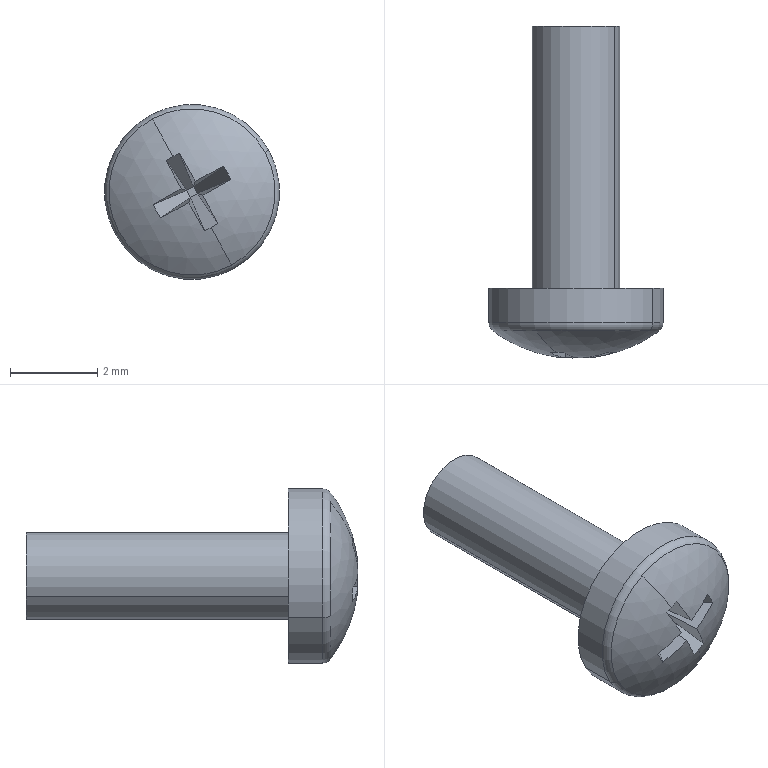Component | SolidWorks | pan cross head_am_pkg-24 | 1 solid | 23 faces | box 4 x 7.59 x 4 mm | volume 34 mm3 | plane 15 | cylinder 4 | torus 2 | sphere 2 | commonest cylinder face diameters 4 x2 2 x2
STEP:
#1=COLOUR_RGB('',0.7922,0.8196,0.9333);
#2=FILL_AREA_STYLE_COLOUR('',#1);
#3=FILL_AREA_STYLE('',(#2));
#4=SURFACE_STYLE_FILL_AREA(#3);
#5=SURFACE_SIDE_STYLE('',(#4));
#6=SURFACE_STYLE_USAGE(.BOTH.,#5);
#7=PRESENTATION_STYLE_ASSIGNMENT((#6));
#8=CARTESIAN_POINT('',(-3.41,0.1268,3.067));
#9=VERTEX_POINT('',#8);
#10=CARTESIAN_POINT('',(-3.271,0.1268,3.142));
#11=VERTEX_POINT('',#10);
#12=CARTESIAN_POINT('',(-3.341,0.1268,3.104));
#13=DIRECTION('',(0.,-1.,0.));
#14=DIRECTION('',(-0.8793,0.,-0.4763));
#15=AXIS2_PLACEMENT_3D('',#12,#13,#14);
#16=CIRCLE('',#15,0.07874);
#17=EDGE_CURVE('',#9,#11,#16,.T.);
#18=ORIENTED_EDGE('',*,*,#17,.T.);
#19=CARTESIAN_POINT('',(-3.275,0.1192,3.14));
#20=VERTEX_POINT('',#19);
#21=CARTESIAN_POINT('',(-3.28,0.1268,3.137));
#22=DIRECTION('',(0.4763,0.,-0.8793));
#23=DIRECTION('',(-0.8793,0.,-0.4763));
#24=AXIS2_PLACEMENT_3D('',#21,#22,#23);
#25=CIRCLE('',#24,0.009449);
#26=EDGE_CURVE('',#11,#20,#25,.T.);
#27=ORIENTED_EDGE('',*,*,#26,.T.);
#28=CARTESIAN_POINT('',(-3.305,0.1192,3.039));
#29=VERTEX_POINT('',#28);
#30=CARTESIAN_POINT('',(-3.341,0.1192,3.104));
#31=DIRECTION('',(0.,-1.,0.));
#32=DIRECTION('',(-0.8793,0.,-0.4763));
#33=AXIS2_PLACEMENT_3D('',#30,#31,#32);
#34=CIRCLE('',#33,0.07491);
#35=EDGE_CURVE('',#29,#20,#34,.T.);
#36=ORIENTED_EDGE('',*,*,#35,.F.);
#37=CARTESIAN_POINT('',(-3.407,0.1192,3.069));
#38=VERTEX_POINT('',#37);
#39=CARTESIAN_POINT('',(-3.341,0.1192,3.104));
#40=DIRECTION('',(0.,-1.,0.));
#41=DIRECTION('',(-0.8793,0.,-0.4763));
#42=AXIS2_PLACEMENT_3D('',#39,#40,#41);
#43=CIRCLE('',#42,0.07491);
#44=EDGE_CURVE('',#38,#29,#43,.T.);
#45=ORIENTED_EDGE('',*,*,#44,.F.);
#46=CARTESIAN_POINT('',(-3.402,0.1268,3.071));
#47=DIRECTION('',(-0.4763,0.,0.8793));
#48=DIRECTION('',(0.8793,0.,0.4763));
#49=AXIS2_PLACEMENT_3D('',#46,#47,#48);
#50=CIRCLE('',#49,0.009449);
#51=EDGE_CURVE('',#9,#38,#50,.T.);
#52=ORIENTED_EDGE('',*,*,#51,.F.);
#53=EDGE_LOOP('',(#18,#27,#36,#45,#52));
#54=FACE_OUTER_BOUND('',#53,.T.);
#55=CARTESIAN_POINT('',(-3.341,0.1268,3.104));
#56=DIRECTION('',(0.,-1.,0.));
#57=DIRECTION('',(-0.8793,0.,-0.4763));
#58=AXIS2_PLACEMENT_3D('',#55,#56,#57);
#59=TOROIDAL_SURFACE('',#58,0.06929,0.009449);
#60=ADVANCED_FACE('',(#54),#59,.T.);
#61=CARTESIAN_POINT('',(-3.41,0.1575,3.067));
#62=VERTEX_POINT('',#61);
#63=CARTESIAN_POINT('',(-3.271,0.1575,3.142));
#64=VERTEX_POINT('',#63);
#65=CARTESIAN_POINT('',(-3.341,0.1575,3.104));
#66=DIRECTION('',(0.,-1.,0.));
#67=DIRECTION('',(-0.8793,0.,-0.4763));
#68=AXIS2_PLACEMENT_3D('',#65,#66,#67);
#69=CIRCLE('',#68,0.07874);
#70=EDGE_CURVE('',#62,#64,#69,.T.);
#71=ORIENTED_EDGE('',*,*,#70,.T.);
#72=CARTESIAN_POINT('',(-3.271,-0.9055,3.142));
#73=DIRECTION('',(0.,-1.,0.));
#74=VECTOR('',#73,39.37);
#75=LINE('',#72,#74);
#76=EDGE_CURVE('',#64,#11,#75,.T.);
#77=ORIENTED_EDGE('',*,*,#76,.T.);
#78=ORIENTED_EDGE('',*,*,#17,.F.);
#79=CARTESIAN_POINT('',(-3.41,-0.9055,3.067));
#80=DIRECTION('',(0.,-1.,0.));
#81=VECTOR('',#80,39.37);
#82=LINE('',#79,#81);
#83=EDGE_CURVE('',#62,#9,#82,.T.);
#84=ORIENTED_EDGE('',*,*,#83,.F.);
#85=EDGE_LOOP('',(#71,#77,#78,#84));
#86=FACE_OUTER_BOUND('',#85,.T.);
#87=CARTESIAN_POINT('',(-3.341,-0.9055,3.104));
#88=DIRECTION('',(0.,-1.,0.));
#89=DIRECTION('',(-0.8793,0.,-0.4763));
#90=AXIS2_PLACEMENT_3D('',#87,#88,#89);
#91=CYLINDRICAL_SURFACE('',#90,0.07874);
#92=ADVANCED_FACE('',(#86),#91,.T.);
#93=CARTESIAN_POINT('',(-3.375,0.3937,3.086));
#94=VERTEX_POINT('',#93);
#95=CARTESIAN_POINT('',(-3.306,0.3937,3.123));
#96=VERTEX_POINT('',#95);
#97=CARTESIAN_POINT('',(-3.341,0.3937,3.104));
#98=DIRECTION('',(0.,-1.,0.));
#99=DIRECTION('',(-0.8793,0.,-0.4763));
#100=AXIS2_PLACEMENT_3D('',#97,#98,#99);
#101=CIRCLE('',#100,0.03937);
#102=EDGE_CURVE('',#94,#96,#101,.T.);
#103=ORIENTED_EDGE('',*,*,#102,.T.);
#104=CARTESIAN_POINT('',(-3.306,0.1575,3.123));
#105=VERTEX_POINT('',#104);
#106=CARTESIAN_POINT('',(-3.306,-0.9055,3.123));
#107=DIRECTION('',(0.,-1.,0.));
#108=VECTOR('',#107,39.37);
#109=LINE('',#106,#108);
#110=EDGE_CURVE('',#96,#105,#109,.T.);
#111=ORIENTED_EDGE('',*,*,#110,.T.);
#112=CARTESIAN_POINT('',(-3.375,0.1575,3.086));
#113=VERTEX_POINT('',#112);
#114=CARTESIAN_POINT('',(-3.341,0.1575,3.104));
#115=DIRECTION('',(0.,-1.,0.));
#116=DIRECTION('',(-0.8793,0.,-0.4763));
#117=AXIS2_PLACEMENT_3D('',#114,#115,#116);
#118=CIRCLE('',#117,0.03937);
#119=EDGE_CURVE('',#113,#105,#118,.T.);
#120=ORIENTED_EDGE('',*,*,#119,.F.);
#121=CARTESIAN_POINT('',(-3.375,-0.9055,3.086));
#122=DIRECTION('',(0.,-1.,0.));
#123=VECTOR('',#122,39.37);
#124=LINE('',#121,#123);
#125=EDGE_CURVE('',#94,#113,#124,.T.);
#126=ORIENTED_EDGE('',*,*,#125,.F.);
#127=EDGE_LOOP('',(#103,#111,#120,#126));
#128=FACE_OUTER_BOUND('',#127,.T.);
#129=CARTESIAN_POINT('',(-3.341,-0.9055,3.104));
#130=DIRECTION('',(0.,-1.,0.));
#131=DIRECTION('',(-0.8793,0.,-0.4763));
#132=AXIS2_PLACEMENT_3D('',#129,#130,#131);
#133=CYLINDRICAL_SURFACE('',#132,0.03937);
#134=ADVANCED_FACE('',(#128),#133,.T.);
#135=ORIENTED_EDGE('',*,*,#35,.T.);
#136=CARTESIAN_POINT('',(-3.376,0.1192,3.17));
#137=VERTEX_POINT('',#136);
#138=CARTESIAN_POINT('',(-3.341,0.1192,3.104));
#139=DIRECTION('',(0.,-1.,0.));
#140=DIRECTION('',(-0.8793,0.,-0.4763));
#141=AXIS2_PLACEMENT_3D('',#138,#139,#140);
#142=CIRCLE('',#141,0.07491);
#143=EDGE_CURVE('',#20,#137,#142,.T.);
#144=ORIENTED_EDGE('',*,*,#143,.T.);
#145=CARTESIAN_POINT('',(-3.358,0.09982,3.136));
#146=VERTEX_POINT('',#145);
#147=CARTESIAN_POINT('',(-3.341,0.2205,3.104));
#148=DIRECTION('',(0.8793,0.,0.4763));
#149=DIRECTION('',(0.4763,0.,-0.8793));
#150=AXIS2_PLACEMENT_3D('',#147,#148,#149);
#151=CIRCLE('',#150,0.126);
#152=EDGE_CURVE('',#137,#146,#151,.T.);
#153=ORIENTED_EDGE('',*,*,#152,.T.);
#154=CARTESIAN_POINT('',(-3.352,0.09998,3.14));
#155=VERTEX_POINT('',#154);
#156=CARTESIAN_POINT('',(-3.325,0.197,3.075));
#157=DIRECTION('',(-0.3878,0.5805,0.716));
#158=DIRECTION('',(0.2765,0.8143,-0.5104));
#159=AXIS2_PLACEMENT_3D('',#156,#157,#158);
#160=CIRCLE('',#159,0.1193);
#161=EDGE_CURVE('',#146,#155,#160,.T.);
#162=ORIENTED_EDGE('',*,*,#161,.T.);
#163=CARTESIAN_POINT('',(-3.338,0.0949,3.114));
#164=VERTEX_POINT('',#163);
#165=CARTESIAN_POINT('',(-3.342,0.2204,3.104));
#166=DIRECTION('',(-0.8771,-0.07065,-0.4751));
#167=DIRECTION('',(-0.06212,0.9975,-0.03365));
#168=AXIS2_PLACEMENT_3D('',#165,#166,#167);
#169=CIRCLE('',#168,0.126);
#170=EDGE_CURVE('',#164,#155,#169,.T.);
#171=ORIENTED_EDGE('',*,*,#170,.F.);
#172=CARTESIAN_POINT('',(-3.312,0.09998,3.128));
#173=VERTEX_POINT('',#172);
#174=CARTESIAN_POINT('',(-3.34,0.2204,3.103));
#175=DIRECTION('',(0.4751,-0.07065,-0.8771));
#176=DIRECTION('',(-0.03365,-0.9975,0.06212));
#177=AXIS2_PLACEMENT_3D('',#174,#175,#176);
#178=CIRCLE('',#177,0.126);
#179=EDGE_CURVE('',#173,#164,#178,.T.);
#180=ORIENTED_EDGE('',*,*,#179,.F.);
#181=CARTESIAN_POINT('',(-3.306,0.09998,3.116));
#182=VERTEX_POINT('',#181);
#183=CARTESIAN_POINT('',(-3.37,0.197,3.089));
#184=DIRECTION('',(0.716,0.5805,0.3878));
#185=DIRECTION('',(0.5104,-0.8143,0.2765));
#186=AXIS2_PLACEMENT_3D('',#183,#184,#185);
#187=CIRCLE('',#186,0.1193);
#188=EDGE_CURVE('',#173,#182,#187,.T.);
#189=ORIENTED_EDGE('',*,*,#188,.T.);
#190=CARTESIAN_POINT('',(-3.331,0.0949,3.102));
#191=VERTEX_POINT('',#190);
#192=CARTESIAN_POINT('',(-3.341,0.2204,3.106));
#193=DIRECTION('',(-0.4751,-0.07065,0.8771));
#194=DIRECTION('',(-0.03365,0.9975,0.06212));
#195=AXIS2_PLACEMENT_3D('',#192,#193,#194);
#196=CIRCLE('',#195,0.126);
#197=EDGE_CURVE('',#191,#182,#196,.T.);
#198=ORIENTED_EDGE('',*,*,#197,.F.);
#199=CARTESIAN_POINT('',(-3.317,0.09998,3.076));
#200=VERTEX_POINT('',#199);
#201=CARTESIAN_POINT('',(-3.342,0.2204,3.104));
#202=DIRECTION('',(-0.8771,-0.07065,-0.4751));
#203=DIRECTION('',(-0.06212,0.9975,-0.03365));
#204=AXIS2_PLACEMENT_3D('',#201,#202,#203);
#205=CIRCLE('',#204,0.126);
#206=EDGE_CURVE('',#200,#191,#205,.T.);
#207=ORIENTED_EDGE('',*,*,#206,.F.);
#208=CARTESIAN_POINT('',(-3.323,0.09982,3.073));
#209=VERTEX_POINT('',#208);
#210=CARTESIAN_POINT('',(-3.356,0.197,3.133));
#211=DIRECTION('',(0.3878,0.5805,-0.716));
#212=DIRECTION('',(0.2765,-0.8143,-0.5104));
#213=AXIS2_PLACEMENT_3D('',#210,#211,#212);
#214=CIRCLE('',#213,0.1193);
#215=EDGE_CURVE('',#200,#209,#214,.T.);
#216=ORIENTED_EDGE('',*,*,#215,.T.);
#217=CARTESIAN_POINT('',(-3.341,0.2205,3.104));
#218=DIRECTION('',(-0.8793,0.,-0.4763));
#219=DIRECTION('',(-0.4763,0.,0.8793));
#220=AXIS2_PLACEMENT_3D('',#217,#218,#219);
#221=CIRCLE('',#220,0.126);
#222=EDGE_CURVE('',#29,#209,#221,.T.);
#223=ORIENTED_EDGE('',*,*,#222,.F.);
#224=EDGE_LOOP('',(#135,#144,#153,#162,#171,#180,#189,#198,#207,#216,#223));
#225=FACE_OUTER_BOUND('',#224,.T.);
#226=CARTESIAN_POINT('',(-3.341,0.2205,3.104));
#227=DIRECTION('',(0.8793,0.,0.4763));
#228=DIRECTION('',(0.4763,0.,-0.8793));
#229=AXIS2_PLACEMENT_3D('',#226,#227,#228);
#230=SPHERICAL_SURFACE('',#229,0.126);
#231=ADVANCED_FACE('',(#225),#230,.T.);
#232=ORIENTED_EDGE('',*,*,#152,.F.);
#233=CARTESIAN_POINT('',(-3.341,0.1192,3.104));
#234=DIRECTION('',(0.,-1.,0.));
#235=DIRECTION('',(-0.8793,0.,-0.4763));
#236=AXIS2_PLACEMENT_3D('',#233,#234,#235);
#237=CIRCLE('',#236,0.07491);
#238=EDGE_CURVE('',#137,#38,#237,.T.);
#239=ORIENTED_EDGE('',*,*,#238,.T.);
#240=ORIENTED_EDGE('',*,*,#44,.T.);
#241=ORIENTED_EDGE('',*,*,#222,.T.);
#242=CARTESIAN_POINT('',(-3.329,0.09998,3.069));
#243=VERTEX_POINT('',#242);
#244=CARTESIAN_POINT('',(-3.356,0.197,3.133));
#245=DIRECTION('',(0.3878,0.5805,-0.716));
#246=DIRECTION('',(0.2765,-0.8143,-0.5104));
#247=AXIS2_PLACEMENT_3D('',#244,#245,#246);
#248=CIRCLE('',#247,0.1193);
#249=EDGE_CURVE('',#209,#243,#248,.T.);
#250=ORIENTED_EDGE('',*,*,#249,.T.);
#251=CARTESIAN_POINT('',(-3.344,0.0949,3.095));
#252=VERTEX_POINT('',#251);
#253=CARTESIAN_POINT('',(-3.339,0.2204,3.105));
#254=DIRECTION('',(0.8771,-0.07065,0.4751));
#255=DIRECTION('',(-0.06212,-0.9975,-0.03365));
#256=AXIS2_PLACEMENT_3D('',#253,#254,#255);
#257=CIRCLE('',#256,0.126);
#258=EDGE_CURVE('',#252,#243,#257,.T.);
#259=ORIENTED_EDGE('',*,*,#258,.F.);
#260=CARTESIAN_POINT('',(-3.369,0.09998,3.081));
#261=VERTEX_POINT('',#260);
#262=CARTESIAN_POINT('',(-3.341,0.2204,3.106));
#263=DIRECTION('',(-0.4751,-0.07065,0.8771));
#264=DIRECTION('',(-0.03365,0.9975,0.06212));
#265=AXIS2_PLACEMENT_3D('',#262,#263,#264);
#266=CIRCLE('',#265,0.126);
#267=EDGE_CURVE('',#261,#252,#266,.T.);
#268=ORIENTED_EDGE('',*,*,#267,.F.);
#269=CARTESIAN_POINT('',(-3.376,0.09998,3.093));
#270=VERTEX_POINT('',#269);
#271=CARTESIAN_POINT('',(-3.312,0.197,3.12));
#272=DIRECTION('',(-0.716,0.5805,-0.3878));
#273=DIRECTION('',(0.5104,0.8143,0.2765));
#274=AXIS2_PLACEMENT_3D('',#271,#272,#273);
#275=CIRCLE('',#274,0.1193);
#276=EDGE_CURVE('',#261,#270,#275,.T.);
#277=ORIENTED_EDGE('',*,*,#276,.T.);
#278=CARTESIAN_POINT('',(-3.35,0.0949,3.107));
#279=VERTEX_POINT('',#278);
#280=CARTESIAN_POINT('',(-3.34,0.2204,3.103));
#281=DIRECTION('',(0.4751,-0.07065,-0.8771));
#282=DIRECTION('',(-0.03365,-0.9975,0.06212));
#283=AXIS2_PLACEMENT_3D('',#280,#281,#282);
#284=CIRCLE('',#283,0.126);
#285=EDGE_CURVE('',#279,#270,#284,.T.);
#286=ORIENTED_EDGE('',*,*,#285,.F.);
#287=CARTESIAN_POINT('',(-3.364,0.09998,3.133));
#288=VERTEX_POINT('',#287);
#289=CARTESIAN_POINT('',(-3.339,0.2204,3.105));
#290=DIRECTION('',(0.8771,-0.07065,0.4751));
#291=DIRECTION('',(-0.06212,-0.9975,-0.03365));
#292=AXIS2_PLACEMENT_3D('',#289,#290,#291);
#293=CIRCLE('',#292,0.126);
#294=EDGE_CURVE('',#288,#279,#293,.T.);
#295=ORIENTED_EDGE('',*,*,#294,.F.);
#296=CARTESIAN_POINT('',(-3.325,0.197,3.075));
#297=DIRECTION('',(-0.3878,0.5805,0.716));
#298=DIRECTION('',(0.2765,0.8143,-0.5104));
#299=AXIS2_PLACEMENT_3D('',#296,#297,#298);
#300=CIRCLE('',#299,0.1193);
#301=EDGE_CURVE('',#288,#146,#300,.T.);
#302=ORIENTED_EDGE('',*,*,#301,.T.);
#303=EDGE_LOOP('',(#232,#239,#240,#241,#250,#259,#268,#277,#286,#295,#302));
#304=FACE_OUTER_BOUND('',#303,.T.);
#305=CARTESIAN_POINT('',(-3.341,0.2205,3.104));
#306=DIRECTION('',(0.8793,0.,0.4763));
#307=DIRECTION('',(0.4763,0.,-0.8793));
#308=AXIS2_PLACEMENT_3D('',#305,#306,#307);
#309=SPHERICAL_SURFACE('',#308,0.126);
#310=ADVANCED_FACE('',(#304),#309,.T.);
#311=ORIENTED_EDGE('',*,*,#206,.T.);
#312=CARTESIAN_POINT('',(-3.336,0.1456,3.103));
#313=VERTEX_POINT('',#312);
#314=CARTESIAN_POINT('',(-3.336,0.1509,3.103));
#315=DIRECTION('',(-0.09553,0.995,0.0284));
#316=VECTOR('',#315,39.37);
#317=LINE('',#314,#316);
#318=EDGE_CURVE('',#191,#313,#317,.T.);
#319=ORIENTED_EDGE('',*,*,#318,.T.);
#320=CARTESIAN_POINT('',(-3.315,0.09449,3.073));
#321=DIRECTION('',(-0.3266,0.8129,0.4821));
#322=VECTOR('',#321,39.37);
#323=LINE('',#320,#322);
#324=EDGE_CURVE('',#200,#313,#323,.T.);
#325=ORIENTED_EDGE('',*,*,#324,.F.);
#326=EDGE_LOOP('',(#311,#319,#325));
#327=FACE_OUTER_BOUND('',#326,.T.);
#328=CARTESIAN_POINT('',(-3.338,0.1507,3.106));
#329=DIRECTION('',(-0.8771,-0.07065,-0.4751));
#330=DIRECTION('',(-0.06212,0.9975,-0.03365));
#331=AXIS2_PLACEMENT_3D('',#328,#329,#330);
#332=PLANE('',#331);
#333=ADVANCED_FACE('',(#327),#332,.T.);
#334=CARTESIAN_POINT('',(-3.339,0.1456,3.109));
#335=VERTEX_POINT('',#334);
#336=CARTESIAN_POINT('',(-3.353,0.09449,3.143));
#337=DIRECTION('',(0.2254,0.8129,-0.537));
#338=VECTOR('',#337,39.37);
#339=LINE('',#336,#338);
#340=EDGE_CURVE('',#155,#335,#339,.T.);
#341=ORIENTED_EDGE('',*,*,#340,.T.);
#342=CARTESIAN_POINT('',(-3.339,0.1509,3.109));
#343=DIRECTION('',(0.0284,-0.995,0.09553));
#344=VECTOR('',#343,39.37);
#345=LINE('',#342,#344);
#346=EDGE_CURVE('',#335,#164,#345,.T.);
#347=ORIENTED_EDGE('',*,*,#346,.T.);
#348=ORIENTED_EDGE('',*,*,#170,.T.);
#349=EDGE_LOOP('',(#341,#347,#348));
#350=FACE_OUTER_BOUND('',#349,.T.);
#351=CARTESIAN_POINT('',(-3.338,0.1507,3.106));
#352=DIRECTION('',(-0.8771,-0.07065,-0.4751));
#353=DIRECTION('',(-0.06212,0.9975,-0.03365));
#354=AXIS2_PLACEMENT_3D('',#351,#352,#353);
#355=PLANE('',#354);
#356=ADVANCED_FACE('',(#350),#355,.T.);
#357=CARTESIAN_POINT('',(-3.342,0.1456,3.1));
#358=VERTEX_POINT('',#357);
#359=CARTESIAN_POINT('',(-3.328,0.09449,3.066));
#360=DIRECTION('',(-0.2254,0.8129,0.537));
#361=VECTOR('',#360,39.37);
#362=LINE('',#359,#361);
#363=EDGE_CURVE('',#243,#358,#362,.T.);
#364=ORIENTED_EDGE('',*,*,#363,.T.);
#365=CARTESIAN_POINT('',(-3.342,0.1509,3.1));
#366=DIRECTION('',(-0.0284,-0.995,-0.09553));
#367=VECTOR('',#366,39.37);
#368=LINE('',#365,#367);
#369=EDGE_CURVE('',#358,#252,#368,.T.);
#370=ORIENTED_EDGE('',*,*,#369,.T.);
#371=ORIENTED_EDGE('',*,*,#258,.T.);
#372=EDGE_LOOP('',(#364,#370,#371));
#373=FACE_OUTER_BOUND('',#372,.T.);
#374=CARTESIAN_POINT('',(-3.344,0.1507,3.103));
#375=DIRECTION('',(0.8771,-0.07065,0.4751));
#376=DIRECTION('',(-0.06212,-0.9975,-0.03365));
#377=AXIS2_PLACEMENT_3D('',#374,#375,#376);
#378=PLANE('',#377);
#379=ADVANCED_FACE('',(#373),#378,.T.);
#380=ORIENTED_EDGE('',*,*,#294,.T.);
#381=CARTESIAN_POINT('',(-3.346,0.1456,3.106));
#382=VERTEX_POINT('',#381);
#383=CARTESIAN_POINT('',(-3.345,0.1509,3.106));
#384=DIRECTION('',(0.09553,0.995,-0.0284));
#385=VECTOR('',#384,39.37);
#386=LINE('',#383,#385);
#387=EDGE_CURVE('',#279,#382,#386,.T.);
#388=ORIENTED_EDGE('',*,*,#387,.T.);
#389=CARTESIAN_POINT('',(-3.366,0.09449,3.136));
#390=DIRECTION('',(0.3266,0.8129,-0.4821));
#391=VECTOR('',#390,39.37);
#392=LINE('',#389,#391);
#393=EDGE_CURVE('',#288,#382,#392,.T.);
#394=ORIENTED_EDGE('',*,*,#393,.F.);
#395=EDGE_LOOP('',(#380,#388,#394));
#396=FACE_OUTER_BOUND('',#395,.T.);
#397=CARTESIAN_POINT('',(-3.344,0.1507,3.103));
#398=DIRECTION('',(0.8771,-0.07065,0.4751));
#399=DIRECTION('',(-0.06212,-0.9975,-0.03365));
#400=AXIS2_PLACEMENT_3D('',#397,#398,#399);
#401=PLANE('',#400);
#402=ADVANCED_FACE('',(#396),#401,.T.);
#403=ORIENTED_EDGE('',*,*,#110,.F.);
#404=CARTESIAN_POINT('',(-3.341,0.3937,3.104));
#405=DIRECTION('',(0.,-1.,0.));
#406=DIRECTION('',(-0.8793,0.,-0.4763));
#407=AXIS2_PLACEMENT_3D('',#404,#405,#406);
#408=CIRCLE('',#407,0.03937);
#409=EDGE_CURVE('',#96,#94,#408,.T.);
#410=ORIENTED_EDGE('',*,*,#409,.T.);
#411=ORIENTED_EDGE('',*,*,#125,.T.);
#412=CARTESIAN_POINT('',(-3.341,0.1575,3.104));
#413=DIRECTION('',(0.,-1.,0.));
#414=DIRECTION('',(-0.8793,0.,-0.4763));
#415=AXIS2_PLACEMENT_3D('',#412,#413,#414);
#416=CIRCLE('',#415,0.03937);
#417=EDGE_CURVE('',#105,#113,#416,.T.);
#418=ORIENTED_EDGE('',*,*,#417,.F.);
#419=EDGE_LOOP('',(#403,#410,#411,#418));
#420=FACE_OUTER_BOUND('',#419,.T.);
#421=CARTESIAN_POINT('',(-3.341,-0.9055,3.104));
#422=DIRECTION('',(0.,-1.,0.));
#423=DIRECTION('',(-0.8793,0.,-0.4763));
#424=AXIS2_PLACEMENT_3D('',#421,#422,#423);
#425=CYLINDRICAL_SURFACE('',#424,0.03937);
#426=ADVANCED_FACE('',(#420),#425,.T.);
#427=ORIENTED_EDGE('',*,*,#70,.F.);
#428=CARTESIAN_POINT('',(-3.341,0.1575,3.104));
#429=DIRECTION('',(0.,-1.,0.));
#430=DIRECTION('',(-0.8793,0.,-0.4763));
#431=AXIS2_PLACEMENT_3D('',#428,#429,#430);
#432=CIRCLE('',#431,0.07874);
#433=EDGE_CURVE('',#64,#62,#432,.T.);
#434=ORIENTED_EDGE('',*,*,#433,.F.);
#435=EDGE_LOOP('',(#427,#434));
#436=FACE_OUTER_BOUND('',#435,.T.);
#437=ORIENTED_EDGE('',*,*,#119,.T.);
#438=ORIENTED_EDGE('',*,*,#417,.T.);
#439=EDGE_LOOP('',(#437,#438));
#440=FACE_BOUND('',#439,.T.);
#441=CARTESIAN_POINT('',(-3.322,0.1575,3.07));
#442=DIRECTION('',(0.,-1.,0.));
#443=DIRECTION('',(-0.8793,0.,-0.4763));
#444=AXIS2_PLACEMENT_3D('',#441,#442,#443);
#445=PLANE('',#444);
#446=ADVANCED_FACE('',(#436,#440),#445,.F.);
#447=ORIENTED_EDGE('',*,*,#76,.F.);
#448=ORIENTED_EDGE('',*,*,#433,.T.);
#449=ORIENTED_EDGE('',*,*,#83,.T.);
#450=CARTESIAN_POINT('',(-3.341,0.1268,3.104));
#451=DIRECTION('',(0.,-1.,0.));
#452=DIRECTION('',(-0.8793,0.,-0.4763));
#453=AXIS2_PLACEMENT_3D('',#450,#451,#452);
#454=CIRCLE('',#453,0.07874);
#455=EDGE_CURVE('',#11,#9,#454,.T.);
#456=ORIENTED_EDGE('',*,*,#455,.F.);
#457=EDGE_LOOP('',(#447,#448,#449,#456));
#458=FACE_OUTER_BOUND('',#457,.T.);
#459=CARTESIAN_POINT('',(-3.341,-0.9055,3.104));
#460=DIRECTION('',(0.,-1.,0.));
#461=DIRECTION('',(-0.8793,0.,-0.4763));
#462=AXIS2_PLACEMENT_3D('',#459,#460,#461);
#463=CYLINDRICAL_SURFACE('',#462,0.07874);
#464=ADVANCED_FACE('',(#458),#463,.T.);
#465=ORIENTED_EDGE('',*,*,#26,.F.);
#466=ORIENTED_EDGE('',*,*,#455,.T.);
#467=ORIENTED_EDGE('',*,*,#51,.T.);
#468=ORIENTED_EDGE('',*,*,#238,.F.);
#469=ORIENTED_EDGE('',*,*,#143,.F.);
#470=EDGE_LOOP('',(#465,#466,#467,#468,#469));
#471=FACE_OUTER_BOUND('',#470,.T.);
#472=CARTESIAN_POINT('',(-3.341,0.1268,3.104));
#473=DIRECTION('',(0.,-1.,0.));
#474=DIRECTION('',(-0.8793,0.,-0.4763));
#475=AXIS2_PLACEMENT_3D('',#472,#473,#474);
#476=TOROIDAL_SURFACE('',#475,0.06929,0.009449);
#477=ADVANCED_FACE('',(#471),#476,.T.);
#478=ORIENTED_EDGE('',*,*,#102,.F.);
#479=ORIENTED_EDGE('',*,*,#409,.F.);
#480=EDGE_LOOP('',(#478,#479));
#481=FACE_OUTER_BOUND('',#480,.T.);
#482=CARTESIAN_POINT('',(-3.322,0.3937,3.07));
#483=DIRECTION('',(0.,1.,0.));
#484=DIRECTION('',(0.8793,0.,0.4763));
#485=AXIS2_PLACEMENT_3D('',#482,#483,#484);
#486=PLANE('',#485);
#487=ADVANCED_FACE('',(#481),#486,.T.);
#488=ORIENTED_EDGE('',*,*,#324,.T.);
#489=CARTESIAN_POINT('',(-3.342,0.1456,3.1));
#490=DIRECTION('',(0.8793,0.,0.4763));
#491=VECTOR('',#490,39.37);
#492=LINE('',#489,#491);
#493=EDGE_CURVE('',#358,#313,#492,.T.);
#494=ORIENTED_EDGE('',*,*,#493,.F.);
#495=ORIENTED_EDGE('',*,*,#363,.F.);
#496=ORIENTED_EDGE('',*,*,#249,.F.);
#497=ORIENTED_EDGE('',*,*,#215,.F.);
#498=EDGE_LOOP('',(#488,#494,#495,#496,#497));
#499=FACE_OUTER_BOUND('',#498,.T.);
#500=CARTESIAN_POINT('',(-3.342,0.1456,3.1));
#501=DIRECTION('',(0.3878,0.5805,-0.716));
#502=DIRECTION('',(0.2765,-0.8143,-0.5104));
#503=AXIS2_PLACEMENT_3D('',#500,#501,#502);
#504=PLANE('',#503);
#505=ADVANCED_FACE('',(#499),#504,.F.);
#506=ORIENTED_EDGE('',*,*,#393,.T.);
#507=CARTESIAN_POINT('',(-3.339,0.1456,3.109));
#508=DIRECTION('',(-0.8793,0.,-0.4763));
#509=VECTOR('',#508,39.37);
#510=LINE('',#507,#509);
#511=EDGE_CURVE('',#335,#382,#510,.T.);
#512=ORIENTED_EDGE('',*,*,#511,.F.);
#513=ORIENTED_EDGE('',*,*,#340,.F.);
#514=ORIENTED_EDGE('',*,*,#161,.F.);
#515=ORIENTED_EDGE('',*,*,#301,.F.);
#516=EDGE_LOOP('',(#506,#512,#513,#514,#515));
#517=FACE_OUTER_BOUND('',#516,.T.);
#518=CARTESIAN_POINT('',(-3.339,0.1456,3.109));
#519=DIRECTION('',(-0.3878,0.5805,0.716));
#520=DIRECTION('',(0.2765,0.8143,-0.5104));
#521=AXIS2_PLACEMENT_3D('',#518,#519,#520);
#522=PLANE('',#521);
#523=ADVANCED_FACE('',(#517),#522,.F.);
#524=CARTESIAN_POINT('',(-3.339,0.1456,3.109));
#525=DIRECTION('',(0.4763,0.,-0.8793));
#526=VECTOR('',#525,39.37);
#527=LINE('',#524,#526);
#528=EDGE_CURVE('',#335,#313,#527,.T.);
#529=ORIENTED_EDGE('',*,*,#528,.F.);
#530=ORIENTED_EDGE('',*,*,#511,.T.);
#531=CARTESIAN_POINT('',(-3.342,0.1456,3.1));
#532=DIRECTION('',(-0.4763,0.,0.8793));
#533=VECTOR('',#532,39.37);
#534=LINE('',#531,#533);
#535=EDGE_CURVE('',#358,#382,#534,.T.);
#536=ORIENTED_EDGE('',*,*,#535,.F.);
#537=ORIENTED_EDGE('',*,*,#493,.T.);
#538=EDGE_LOOP('',(#529,#530,#536,#537));
#539=FACE_OUTER_BOUND('',#538,.T.);
#540=CARTESIAN_POINT('',(-3.336,0.1456,3.103));
#541=DIRECTION('',(0.,-1.,0.));
#542=DIRECTION('',(-0.8793,0.,-0.4763));
#543=AXIS2_PLACEMENT_3D('',#540,#541,#542);
#544=PLANE('',#543);
#545=ADVANCED_FACE('',(#539),#544,.T.);
#546=CARTESIAN_POINT('',(-3.309,0.09449,3.13));
#547=DIRECTION('',(-0.4821,0.8129,-0.3266));
#548=VECTOR('',#547,39.37);
#549=LINE('',#546,#548);
#550=EDGE_CURVE('',#173,#335,#549,.T.);
#551=ORIENTED_EDGE('',*,*,#550,.T.);
#552=ORIENTED_EDGE('',*,*,#528,.T.);
#553=CARTESIAN_POINT('',(-3.302,0.09449,3.117));
#554=DIRECTION('',(-0.537,0.8129,-0.2254));
#555=VECTOR('',#554,39.37);
#556=LINE('',#553,#555);
#557=EDGE_CURVE('',#182,#313,#556,.T.);
#558=ORIENTED_EDGE('',*,*,#557,.F.);
#559=ORIENTED_EDGE('',*,*,#188,.F.);
#560=EDGE_LOOP('',(#551,#552,#558,#559));
#561=FACE_OUTER_BOUND('',#560,.T.);
#562=CARTESIAN_POINT('',(-3.336,0.1456,3.103));
#563=DIRECTION('',(0.716,0.5805,0.3878));
#564=DIRECTION('',(-0.5104,0.8143,-0.2765));
#565=AXIS2_PLACEMENT_3D('',#562,#563,#564);
#566=PLANE('',#565);
#567=ADVANCED_FACE('',(#561),#566,.F.);
#568=ORIENTED_EDGE('',*,*,#179,.T.);
#569=ORIENTED_EDGE('',*,*,#346,.F.);
#570=ORIENTED_EDGE('',*,*,#550,.F.);
#571=EDGE_LOOP('',(#568,#569,#570));
#572=FACE_OUTER_BOUND('',#571,.T.);
#573=CARTESIAN_POINT('',(-3.342,0.1507,3.107));
#574=DIRECTION('',(0.4751,-0.07065,-0.8771));
#575=DIRECTION('',(-0.03365,-0.9975,0.06212));
#576=AXIS2_PLACEMENT_3D('',#573,#574,#575);
#577=PLANE('',#576);
#578=ADVANCED_FACE('',(#572),#577,.T.);
#579=ORIENTED_EDGE('',*,*,#197,.T.);
#580=ORIENTED_EDGE('',*,*,#557,.T.);
#581=ORIENTED_EDGE('',*,*,#318,.F.);
#582=EDGE_LOOP('',(#579,#580,#581));
#583=FACE_OUTER_BOUND('',#582,.T.);
#584=CARTESIAN_POINT('',(-3.339,0.1507,3.102));
#585=DIRECTION('',(-0.4751,-0.07065,0.8771));
#586=DIRECTION('',(-0.03365,0.9975,0.06212));
#587=AXIS2_PLACEMENT_3D('',#584,#585,#586);
#588=PLANE('',#587);
#589=ADVANCED_FACE('',(#583),#588,.T.);
#590=CARTESIAN_POINT('',(-3.372,0.09449,3.079));
#591=DIRECTION('',(0.4821,0.8129,0.3266));
#592=VECTOR('',#591,39.37);
#593=LINE('',#590,#592);
#594=EDGE_CURVE('',#261,#358,#593,.T.);
#595=ORIENTED_EDGE('',*,*,#594,.T.);
#596=ORIENTED_EDGE('',*,*,#535,.T.);
#597=CARTESIAN_POINT('',(-3.379,0.09449,3.092));
#598=DIRECTION('',(0.537,0.8129,0.2254));
#599=VECTOR('',#598,39.37);
#600=LINE('',#597,#599);
#601=EDGE_CURVE('',#270,#382,#600,.T.);
#602=ORIENTED_EDGE('',*,*,#601,.F.);
#603=ORIENTED_EDGE('',*,*,#276,.F.);
#604=EDGE_LOOP('',(#595,#596,#602,#603));
#605=FACE_OUTER_BOUND('',#604,.T.);
#606=CARTESIAN_POINT('',(-3.346,0.1456,3.106));
#607=DIRECTION('',(-0.716,0.5805,-0.3878));
#608=DIRECTION('',(-0.5104,-0.8143,-0.2765));
#609=AXIS2_PLACEMENT_3D('',#606,#607,#608);
#610=PLANE('',#609);
#611=ADVANCED_FACE('',(#605),#610,.F.);
#612=ORIENTED_EDGE('',*,*,#267,.T.);
#613=ORIENTED_EDGE('',*,*,#369,.F.);
#614=ORIENTED_EDGE('',*,*,#594,.F.);
#615=EDGE_LOOP('',(#612,#613,#614));
#616=FACE_OUTER_BOUND('',#615,.T.);
#617=CARTESIAN_POINT('',(-3.339,0.1507,3.102));
#618=DIRECTION('',(-0.4751,-0.07065,0.8771));
#619=DIRECTION('',(-0.03365,0.9975,0.06212));
#620=AXIS2_PLACEMENT_3D('',#617,#618,#619);
#621=PLANE('',#620);
#622=ADVANCED_FACE('',(#616),#621,.T.);
#623=ORIENTED_EDGE('',*,*,#285,.T.);
#624=ORIENTED_EDGE('',*,*,#601,.T.);
#625=ORIENTED_EDGE('',*,*,#387,.F.);
#626=EDGE_LOOP('',(#623,#624,#625));
#627=FACE_OUTER_BOUND('',#626,.T.);
#628=CARTESIAN_POINT('',(-3.342,0.1507,3.107));
#629=DIRECTION('',(0.4751,-0.07065,-0.8771));
#630=DIRECTION('',(-0.03365,-0.9975,0.06212));
#631=AXIS2_PLACEMENT_3D('',#628,#629,#630);
#632=PLANE('',#631);
#633=ADVANCED_FACE('',(#627),#632,.T.);
#634=CLOSED_SHELL('',(#60,#92,#134,#231,#310,#333,#356,#379,#402,#426,#446,#464,#477,#487,#505,#523,#545,#567,#578,#589,#611,#622,#633));
#635=MANIFOLD_SOLID_BREP('',#634);
#636=STYLED_ITEM('',(#7),#635);
#637=(LENGTH_UNIT()NAMED_UNIT(*)SI_UNIT($,.METRE.));
#638=LENGTH_MEASURE_WITH_UNIT(LENGTH_MEASURE(0.0254),#637);
#639=DIMENSIONAL_EXPONENTS(1.,0.,0.,0.,0.,0.,0.);
#640=(CONVERSION_BASED_UNIT('',#638)LENGTH_UNIT()NAMED_UNIT(#639));
#641=UNCERTAINTY_MEASURE_WITH_UNIT(LENGTH_MEASURE(0.00001),#640,'','');
#642=(NAMED_UNIT(*)PLANE_ANGLE_UNIT()SI_UNIT($,.RADIAN.));
#643=(NAMED_UNIT(*)SI_UNIT($,.STERADIAN.)SOLID_ANGLE_UNIT());
#644=(GEOMETRIC_REPRESENTATION_CONTEXT(3)GLOBAL_UNCERTAINTY_ASSIGNED_CONTEXT((#641))GLOBAL_UNIT_ASSIGNED_CONTEXT((#640,#642,#643))REPRESENTATION_CONTEXT('',''));
#645=MECHANICAL_DESIGN_GEOMETRIC_PRESENTATION_REPRESENTATION('',(#636),#644);
#646=CARTESIAN_POINT('',(0.,0.,0.));
#647=DIRECTION('',(0.,0.,1.));
#648=DIRECTION('',(1.,0.,0.));
#649=AXIS2_PLACEMENT_3D('',#646,#647,#648);
#650=(LENGTH_UNIT()NAMED_UNIT(*)SI_UNIT($,.METRE.));
#651=LENGTH_MEASURE_WITH_UNIT(LENGTH_MEASURE(0.0254),#650);
#652=DIMENSIONAL_EXPONENTS(1.,0.,0.,0.,0.,0.,0.);
#653=(CONVERSION_BASED_UNIT('',#651)LENGTH_UNIT()NAMED_UNIT(#652));
#654=UNCERTAINTY_MEASURE_WITH_UNIT(LENGTH_MEASURE(0.00001),#653,'','');
#655=(NAMED_UNIT(*)PLANE_ANGLE_UNIT()SI_UNIT($,.RADIAN.));
#656=(NAMED_UNIT(*)SI_UNIT($,.STERADIAN.)SOLID_ANGLE_UNIT());
#657=(GEOMETRIC_REPRESENTATION_CONTEXT(3)GLOBAL_UNCERTAINTY_ASSIGNED_CONTEXT((#654))GLOBAL_UNIT_ASSIGNED_CONTEXT((#653,#655,#656))REPRESENTATION_CONTEXT('',''));
#658=ADVANCED_BREP_SHAPE_REPRESENTATION('',(#635,#649),#657);
#659=PRESENTATION_LAYER_ASSIGNMENT('','',(#636));